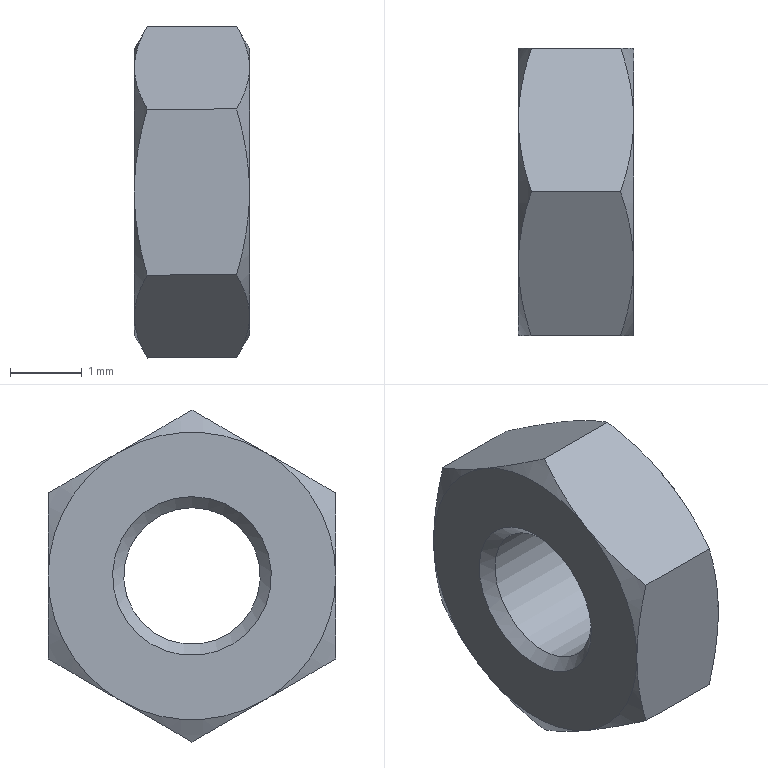Component | NX | GB-T6170_F-2000_M2X0_4 | 1 solid | 23 faces | volume 17 mm3 | cone 14 | plane 8 | cylinder 1 | commonest cylinder face diameters 1.9 x1